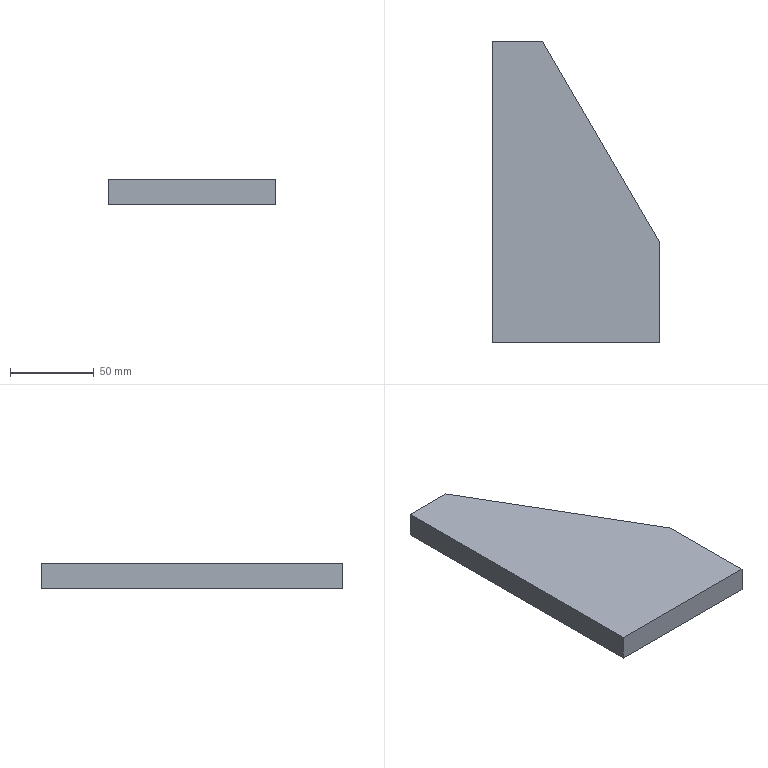Component | SolidWorks | JF21-80.1-1-3(_)-1-SOLID39-1 | 1 solid | 7 faces | box 100 x 180 x 15 mm | volume 207000 mm3 | plane 7
STEP:
#1=COLOUR_RGB('',0.7922,0.8196,0.9333);
#2=FILL_AREA_STYLE_COLOUR('',#1);
#3=FILL_AREA_STYLE('',(#2));
#4=SURFACE_STYLE_FILL_AREA(#3);
#5=SURFACE_SIDE_STYLE('',(#4));
#6=SURFACE_STYLE_USAGE(.BOTH.,#5);
#7=PRESENTATION_STYLE_ASSIGNMENT((#6));
#8=CARTESIAN_POINT('',(21.26,-88.583,40.748));
#9=VERTEX_POINT('',#8);
#10=CARTESIAN_POINT('',(21.26,-86.22,40.748));
#11=VERTEX_POINT('',#10);
#12=CARTESIAN_POINT('',(21.26,-86.22,40.748));
#13=DIRECTION('',(0.,1.,0.));
#14=VECTOR('',#13,39.37);
#15=LINE('',#12,#14);
#16=EDGE_CURVE('',#9,#11,#15,.T.);
#17=ORIENTED_EDGE('',*,*,#16,.F.);
#18=CARTESIAN_POINT('',(21.26,-88.583,40.157));
#19=VERTEX_POINT('',#18);
#20=CARTESIAN_POINT('',(21.26,-88.583,40.157));
#21=DIRECTION('',(0.,0.,1.));
#22=VECTOR('',#21,39.37);
#23=LINE('',#20,#22);
#24=EDGE_CURVE('',#19,#9,#23,.T.);
#25=ORIENTED_EDGE('',*,*,#24,.F.);
#26=CARTESIAN_POINT('',(21.26,-86.22,40.157));
#27=VERTEX_POINT('',#26);
#28=CARTESIAN_POINT('',(21.26,-86.22,40.157));
#29=DIRECTION('',(0.,1.,0.));
#30=VECTOR('',#29,39.37);
#31=LINE('',#28,#30);
#32=EDGE_CURVE('',#19,#27,#31,.T.);
#33=ORIENTED_EDGE('',*,*,#32,.T.);
#34=CARTESIAN_POINT('',(21.26,-86.22,40.157));
#35=DIRECTION('',(0.,0.,1.));
#36=VECTOR('',#35,39.37);
#37=LINE('',#34,#36);
#38=EDGE_CURVE('',#27,#11,#37,.T.);
#39=ORIENTED_EDGE('',*,*,#38,.T.);
#40=EDGE_LOOP('',(#17,#25,#33,#39));
#41=FACE_OUTER_BOUND('',#40,.T.);
#42=CARTESIAN_POINT('',(21.26,-86.22,40.157));
#43=DIRECTION('',(1.,0.,0.));
#44=DIRECTION('',(0.,0.,1.));
#45=AXIS2_PLACEMENT_3D('',#42,#43,#44);
#46=PLANE('',#45);
#47=ADVANCED_FACE('',(#41),#46,.T.);
#48=CARTESIAN_POINT('',(17.323,-88.583,40.748));
#49=VERTEX_POINT('',#48);
#50=CARTESIAN_POINT('',(21.26,-88.583,40.748));
#51=DIRECTION('',(1.,0.,0.));
#52=VECTOR('',#51,39.37);
#53=LINE('',#50,#52);
#54=EDGE_CURVE('',#49,#9,#53,.T.);
#55=ORIENTED_EDGE('',*,*,#54,.F.);
#56=CARTESIAN_POINT('',(17.323,-88.583,40.157));
#57=VERTEX_POINT('',#56);
#58=CARTESIAN_POINT('',(17.323,-88.583,40.157));
#59=DIRECTION('',(0.,0.,1.));
#60=VECTOR('',#59,39.37);
#61=LINE('',#58,#60);
#62=EDGE_CURVE('',#57,#49,#61,.T.);
#63=ORIENTED_EDGE('',*,*,#62,.F.);
#64=CARTESIAN_POINT('',(21.26,-88.583,40.157));
#65=DIRECTION('',(1.,0.,0.));
#66=VECTOR('',#65,39.37);
#67=LINE('',#64,#66);
#68=EDGE_CURVE('',#57,#19,#67,.T.);
#69=ORIENTED_EDGE('',*,*,#68,.T.);
#70=ORIENTED_EDGE('',*,*,#24,.T.);
#71=EDGE_LOOP('',(#55,#63,#69,#70));
#72=FACE_OUTER_BOUND('',#71,.T.);
#73=CARTESIAN_POINT('',(21.26,-88.583,40.157));
#74=DIRECTION('',(0.,-1.,0.));
#75=DIRECTION('',(0.,0.,1.));
#76=AXIS2_PLACEMENT_3D('',#73,#74,#75);
#77=PLANE('',#76);
#78=ADVANCED_FACE('',(#72),#77,.T.);
#79=CARTESIAN_POINT('',(17.323,-81.496,40.748));
#80=VERTEX_POINT('',#79);
#81=CARTESIAN_POINT('',(17.323,-88.583,40.748));
#82=DIRECTION('',(0.,-1.,0.));
#83=VECTOR('',#82,39.37);
#84=LINE('',#81,#83);
#85=EDGE_CURVE('',#80,#49,#84,.T.);
#86=ORIENTED_EDGE('',*,*,#85,.F.);
#87=CARTESIAN_POINT('',(17.323,-81.496,40.157));
#88=VERTEX_POINT('',#87);
#89=CARTESIAN_POINT('',(17.323,-81.496,40.157));
#90=DIRECTION('',(0.,0.,1.));
#91=VECTOR('',#90,39.37);
#92=LINE('',#89,#91);
#93=EDGE_CURVE('',#88,#80,#92,.T.);
#94=ORIENTED_EDGE('',*,*,#93,.F.);
#95=CARTESIAN_POINT('',(17.323,-88.583,40.157));
#96=DIRECTION('',(0.,-1.,0.));
#97=VECTOR('',#96,39.37);
#98=LINE('',#95,#97);
#99=EDGE_CURVE('',#88,#57,#98,.T.);
#100=ORIENTED_EDGE('',*,*,#99,.T.);
#101=ORIENTED_EDGE('',*,*,#62,.T.);
#102=EDGE_LOOP('',(#86,#94,#100,#101));
#103=FACE_OUTER_BOUND('',#102,.T.);
#104=CARTESIAN_POINT('',(17.323,-88.583,40.157));
#105=DIRECTION('',(-1.,0.,0.));
#106=DIRECTION('',(0.,0.,-1.));
#107=AXIS2_PLACEMENT_3D('',#104,#105,#106);
#108=PLANE('',#107);
#109=ADVANCED_FACE('',(#103),#108,.T.);
#110=CARTESIAN_POINT('',(18.504,-81.496,40.748));
#111=VERTEX_POINT('',#110);
#112=CARTESIAN_POINT('',(17.323,-81.496,40.748));
#113=DIRECTION('',(-1.,0.,0.));
#114=VECTOR('',#113,39.37);
#115=LINE('',#112,#114);
#116=EDGE_CURVE('',#111,#80,#115,.T.);
#117=ORIENTED_EDGE('',*,*,#116,.F.);
#118=CARTESIAN_POINT('',(18.504,-81.496,40.157));
#119=VERTEX_POINT('',#118);
#120=CARTESIAN_POINT('',(18.504,-81.496,40.157));
#121=DIRECTION('',(0.,0.,1.));
#122=VECTOR('',#121,39.37);
#123=LINE('',#120,#122);
#124=EDGE_CURVE('',#119,#111,#123,.T.);
#125=ORIENTED_EDGE('',*,*,#124,.F.);
#126=CARTESIAN_POINT('',(17.323,-81.496,40.157));
#127=DIRECTION('',(-1.,0.,0.));
#128=VECTOR('',#127,39.37);
#129=LINE('',#126,#128);
#130=EDGE_CURVE('',#119,#88,#129,.T.);
#131=ORIENTED_EDGE('',*,*,#130,.T.);
#132=ORIENTED_EDGE('',*,*,#93,.T.);
#133=EDGE_LOOP('',(#117,#125,#131,#132));
#134=FACE_OUTER_BOUND('',#133,.T.);
#135=CARTESIAN_POINT('',(17.323,-81.496,40.157));
#136=DIRECTION('',(0.,1.,0.));
#137=DIRECTION('',(0.,0.,-1.));
#138=AXIS2_PLACEMENT_3D('',#135,#136,#137);
#139=PLANE('',#138);
#140=ADVANCED_FACE('',(#134),#139,.T.);
#141=CARTESIAN_POINT('',(18.504,-81.496,40.748));
#142=DIRECTION('',(-0.5039,0.8638,0.));
#143=VECTOR('',#142,39.37);
#144=LINE('',#141,#143);
#145=EDGE_CURVE('',#11,#111,#144,.T.);
#146=ORIENTED_EDGE('',*,*,#145,.F.);
#147=ORIENTED_EDGE('',*,*,#38,.F.);
#148=CARTESIAN_POINT('',(18.504,-81.496,40.157));
#149=DIRECTION('',(-0.5039,0.8638,0.));
#150=VECTOR('',#149,39.37);
#151=LINE('',#148,#150);
#152=EDGE_CURVE('',#27,#119,#151,.T.);
#153=ORIENTED_EDGE('',*,*,#152,.T.);
#154=ORIENTED_EDGE('',*,*,#124,.T.);
#155=EDGE_LOOP('',(#146,#147,#153,#154));
#156=FACE_OUTER_BOUND('',#155,.T.);
#157=CARTESIAN_POINT('',(18.504,-81.496,40.157));
#158=DIRECTION('',(0.8638,0.5039,0.));
#159=DIRECTION('',(0.5039,-0.8638,0.));
#160=AXIS2_PLACEMENT_3D('',#157,#158,#159);
#161=PLANE('',#160);
#162=ADVANCED_FACE('',(#156),#161,.T.);
#163=ORIENTED_EDGE('',*,*,#32,.F.);
#164=ORIENTED_EDGE('',*,*,#68,.F.);
#165=ORIENTED_EDGE('',*,*,#99,.F.);
#166=ORIENTED_EDGE('',*,*,#130,.F.);
#167=ORIENTED_EDGE('',*,*,#152,.F.);
#168=EDGE_LOOP('',(#163,#164,#165,#166,#167));
#169=FACE_OUTER_BOUND('',#168,.T.);
#170=CARTESIAN_POINT('',(21.26,-88.583,40.157));
#171=DIRECTION('',(0.,0.,-1.));
#172=DIRECTION('',(1.,0.,0.));
#173=AXIS2_PLACEMENT_3D('',#170,#171,#172);
#174=PLANE('',#173);
#175=ADVANCED_FACE('',(#169),#174,.T.);
#176=ORIENTED_EDGE('',*,*,#16,.T.);
#177=ORIENTED_EDGE('',*,*,#145,.T.);
#178=ORIENTED_EDGE('',*,*,#116,.T.);
#179=ORIENTED_EDGE('',*,*,#85,.T.);
#180=ORIENTED_EDGE('',*,*,#54,.T.);
#181=EDGE_LOOP('',(#176,#177,#178,#179,#180));
#182=FACE_OUTER_BOUND('',#181,.T.);
#183=CARTESIAN_POINT('',(21.26,-88.583,40.748));
#184=DIRECTION('',(0.,0.,-1.));
#185=DIRECTION('',(1.,0.,0.));
#186=AXIS2_PLACEMENT_3D('',#183,#184,#185);
#187=PLANE('',#186);
#188=ADVANCED_FACE('',(#182),#187,.F.);
#189=CLOSED_SHELL('',(#47,#78,#109,#140,#162,#175,#188));
#190=MANIFOLD_SOLID_BREP('',#189);
#191=STYLED_ITEM('',(#7),#190);
#192=PRESENTATION_LAYER_ASSIGNMENT('','',(#191));
#193=(LENGTH_UNIT()NAMED_UNIT(*)SI_UNIT($,.METRE.));
#194=LENGTH_MEASURE_WITH_UNIT(LENGTH_MEASURE(0.0254),#193);
#195=DIMENSIONAL_EXPONENTS(1.,0.,0.,0.,0.,0.,0.);
#196=(CONVERSION_BASED_UNIT('',#194)LENGTH_UNIT()NAMED_UNIT(#195));
#197=UNCERTAINTY_MEASURE_WITH_UNIT(LENGTH_MEASURE(0.00001),#196,'','');
#198=(NAMED_UNIT(*)PLANE_ANGLE_UNIT()SI_UNIT($,.RADIAN.));
#199=(NAMED_UNIT(*)SI_UNIT($,.STERADIAN.)SOLID_ANGLE_UNIT());
#200=(GEOMETRIC_REPRESENTATION_CONTEXT(3)GLOBAL_UNCERTAINTY_ASSIGNED_CONTEXT((#197))GLOBAL_UNIT_ASSIGNED_CONTEXT((#196,#198,#199))REPRESENTATION_CONTEXT('',''));
#201=MECHANICAL_DESIGN_GEOMETRIC_PRESENTATION_REPRESENTATION('',(#191),#200);
#202=CARTESIAN_POINT('',(0.,0.,0.));
#203=DIRECTION('',(0.,0.,1.));
#204=DIRECTION('',(1.,0.,0.));
#205=AXIS2_PLACEMENT_3D('',#202,#203,#204);
#206=(LENGTH_UNIT()NAMED_UNIT(*)SI_UNIT($,.METRE.));
#207=LENGTH_MEASURE_WITH_UNIT(LENGTH_MEASURE(0.0254),#206);
#208=DIMENSIONAL_EXPONENTS(1.,0.,0.,0.,0.,0.,0.);
#209=(CONVERSION_BASED_UNIT('',#207)LENGTH_UNIT()NAMED_UNIT(#208));
#210=UNCERTAINTY_MEASURE_WITH_UNIT(LENGTH_MEASURE(0.00001),#209,'','');
#211=(NAMED_UNIT(*)PLANE_ANGLE_UNIT()SI_UNIT($,.RADIAN.));
#212=(NAMED_UNIT(*)SI_UNIT($,.STERADIAN.)SOLID_ANGLE_UNIT());
#213=(GEOMETRIC_REPRESENTATION_CONTEXT(3)GLOBAL_UNCERTAINTY_ASSIGNED_CONTEXT((#210))GLOBAL_UNIT_ASSIGNED_CONTEXT((#209,#211,#212))REPRESENTATION_CONTEXT('',''));
#214=ADVANCED_BREP_SHAPE_REPRESENTATION('',(#190,#205),#213);